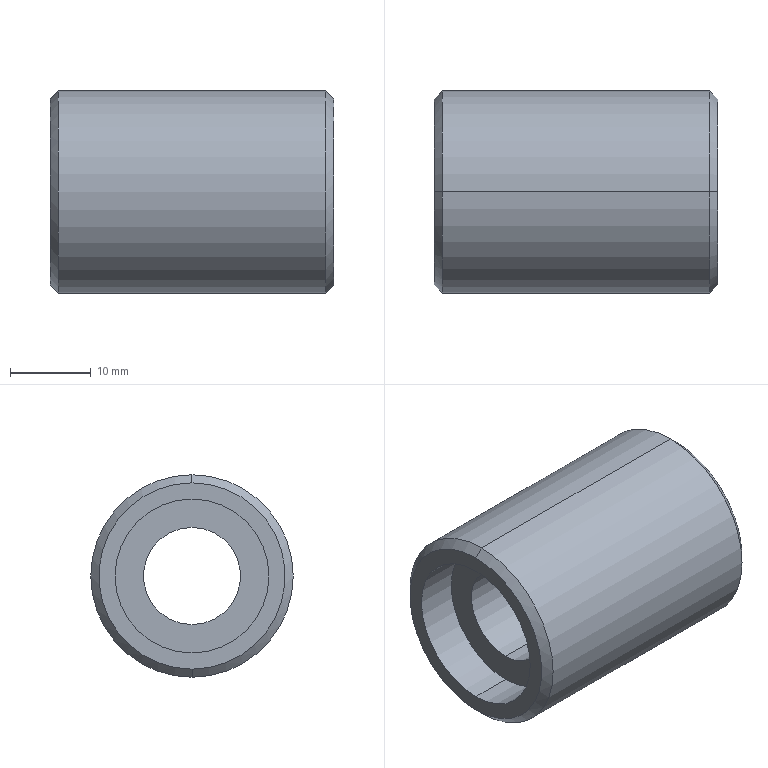Component | SolidWorks | CHEN123-AA-14-2 | 1 solid | 16 faces | box 35 x 25 x 25 mm | volume 11373 mm3 | cylinder 8 | cone 4 | plane 4 | commonest cylinder face diameters 19 x4 25 x2 12 x2
build123d program:
from build123d import *

# Parameters (mm, degrees)
SKETCH1_R           = 12.5
BOSS_EXTRUDE1_DEPTH = 17.5
SKETCH2_R           = 6
CUT_EXTRUDE1_DEPTH  = 40.211
SKETCH3_R           = 9.5
CUT_EXTRUDE2_DEPTH  = 5.2
CUT_EXTRUDE3_START  = -5.2
SKETCH4_R           = 9.5
CUT_EXTRUDE3_DEPTH  = 5.2
CHAMFER1_SIZE       = 1


with BuildPart() as part:
    # Sketch1 → Boss-Extrude1 (new, symmetric)
    with BuildSketch(Plane.XY):
        Circle(SKETCH1_R)
    extrude(amount=BOSS_EXTRUDE1_DEPTH, both=True)

    # Sketch2 → Cut-Extrude1 (cut, through all)
    with BuildSketch(Plane.XY.offset(17.5)):
        Circle(SKETCH2_R)
    extrude(amount=-CUT_EXTRUDE1_DEPTH, mode=Mode.SUBTRACT)

    # Sketch3 → Cut-Extrude2 (cut)
    with BuildSketch(Plane.XY.offset(17.5)):
        Circle(SKETCH3_R)
    extrude(amount=-CUT_EXTRUDE2_DEPTH, mode=Mode.SUBTRACT)

    # Sketch4 → Cut-Extrude3 (cut)
    with BuildSketch(Plane(origin=(0, 0, -17.5), x_dir=(-1, 0, 0), z_dir=(0, 0, -1)).offset(CUT_EXTRUDE3_START)):
        with Locations(Location((0, 0, 0), (0, 0, 180))):
            Circle(SKETCH4_R)
    extrude(amount=CUT_EXTRUDE3_DEPTH, mode=Mode.SUBTRACT)

    # Chamfer1
    chamfer1_edges = [part.edges().sort_by_distance(p)[0] for p in [
        (-12.5, 0, -17.5),
        (-12.5, 0, 17.5),
    ]]
    chamfer(chamfer1_edges, length=CHAMFER1_SIZE)


solid = part.part

# Placed as in the assembly
solid = solid.moved(Location((-0.0005, -45.999, -172), (0, 90, 0)))
STEP:
#1=COLOUR_RGB('',0.7922,0.8196,0.9333);
#2=FILL_AREA_STYLE_COLOUR('',#1);
#3=FILL_AREA_STYLE('',(#2));
#4=SURFACE_STYLE_FILL_AREA(#3);
#5=SURFACE_SIDE_STYLE('',(#4));
#6=SURFACE_STYLE_USAGE(.BOTH.,#5);
#7=PRESENTATION_STYLE_ASSIGNMENT((#6));
#8=CARTESIAN_POINT('',(0.689,-1.811,-7.224));
#9=VERTEX_POINT('',#8);
#10=CARTESIAN_POINT('',(0.689,-1.811,-6.319));
#11=VERTEX_POINT('',#10);
#12=CARTESIAN_POINT('',(0.689,-1.811,-6.772));
#13=DIRECTION('',(1.,0.,0.));
#14=DIRECTION('',(0.,0.,1.));
#15=AXIS2_PLACEMENT_3D('',#12,#13,#14);
#16=CIRCLE('',#15,0.4528);
#17=EDGE_CURVE('',#9,#11,#16,.T.);
#18=ORIENTED_EDGE('',*,*,#17,.F.);
#19=CARTESIAN_POINT('',(0.6496,-1.811,-7.264));
#20=VERTEX_POINT('',#19);
#21=CARTESIAN_POINT('',(0.6496,-1.811,-7.264));
#22=DIRECTION('',(-0.7071,-0.,-0.7071));
#23=VECTOR('',#22,39.37);
#24=LINE('',#21,#23);
#25=EDGE_CURVE('',#9,#20,#24,.T.);
#26=ORIENTED_EDGE('',*,*,#25,.T.);
#27=CARTESIAN_POINT('',(0.6496,-1.811,-6.28));
#28=VERTEX_POINT('',#27);
#29=CARTESIAN_POINT('',(0.6496,-1.811,-6.772));
#30=DIRECTION('',(-1.,0.,0.));
#31=DIRECTION('',(0.,0.,1.));
#32=AXIS2_PLACEMENT_3D('',#29,#30,#31);
#33=CIRCLE('',#32,0.4921);
#34=EDGE_CURVE('',#28,#20,#33,.T.);
#35=ORIENTED_EDGE('',*,*,#34,.F.);
#36=CARTESIAN_POINT('',(0.6496,-1.811,-6.28));
#37=DIRECTION('',(-0.7071,0.,0.7071));
#38=VECTOR('',#37,39.37);
#39=LINE('',#36,#38);
#40=EDGE_CURVE('',#11,#28,#39,.T.);
#41=ORIENTED_EDGE('',*,*,#40,.F.);
#42=EDGE_LOOP('',(#18,#26,#35,#41));
#43=FACE_OUTER_BOUND('',#42,.T.);
#44=CARTESIAN_POINT('',(0.6496,-1.811,-6.772));
#45=DIRECTION('',(-1.,0.,0.));
#46=DIRECTION('',(0.,0.,1.));
#47=AXIS2_PLACEMENT_3D('',#44,#45,#46);
#48=CONICAL_SURFACE('',#47,0.4921,0.7854);
#49=ADVANCED_FACE('',(#43),#48,.T.);
#50=CARTESIAN_POINT('',(-0.689,-1.811,-6.319));
#51=VERTEX_POINT('',#50);
#52=CARTESIAN_POINT('',(-0.689,-1.811,-7.224));
#53=VERTEX_POINT('',#52);
#54=CARTESIAN_POINT('',(-0.689,-1.811,-6.772));
#55=DIRECTION('',(-1.,0.,0.));
#56=DIRECTION('',(0.,0.,1.));
#57=AXIS2_PLACEMENT_3D('',#54,#55,#56);
#58=CIRCLE('',#57,0.4528);
#59=EDGE_CURVE('',#51,#53,#58,.T.);
#60=ORIENTED_EDGE('',*,*,#59,.F.);
#61=CARTESIAN_POINT('',(-0.6496,-1.811,-6.28));
#62=VERTEX_POINT('',#61);
#63=CARTESIAN_POINT('',(-0.689,-1.811,-6.319));
#64=DIRECTION('',(0.7071,0.,0.7071));
#65=VECTOR('',#64,39.37);
#66=LINE('',#63,#65);
#67=EDGE_CURVE('',#51,#62,#66,.T.);
#68=ORIENTED_EDGE('',*,*,#67,.T.);
#69=CARTESIAN_POINT('',(-0.6496,-1.811,-7.264));
#70=VERTEX_POINT('',#69);
#71=CARTESIAN_POINT('',(-0.6496,-1.811,-6.772));
#72=DIRECTION('',(1.,0.,0.));
#73=DIRECTION('',(0.,0.,1.));
#74=AXIS2_PLACEMENT_3D('',#71,#72,#73);
#75=CIRCLE('',#74,0.4921);
#76=EDGE_CURVE('',#70,#62,#75,.T.);
#77=ORIENTED_EDGE('',*,*,#76,.F.);
#78=CARTESIAN_POINT('',(-0.689,-1.811,-7.224));
#79=DIRECTION('',(0.7071,-0.,-0.7071));
#80=VECTOR('',#79,39.37);
#81=LINE('',#78,#80);
#82=EDGE_CURVE('',#53,#70,#81,.T.);
#83=ORIENTED_EDGE('',*,*,#82,.F.);
#84=EDGE_LOOP('',(#60,#68,#77,#83));
#85=FACE_OUTER_BOUND('',#84,.T.);
#86=CARTESIAN_POINT('',(-0.689,-1.811,-6.772));
#87=DIRECTION('',(1.,0.,0.));
#88=DIRECTION('',(0.,-0.,-1.));
#89=AXIS2_PLACEMENT_3D('',#86,#87,#88);
#90=CONICAL_SURFACE('',#89,0.4528,0.7854);
#91=ADVANCED_FACE('',(#85),#90,.T.);
#92=CARTESIAN_POINT('',(0.4842,-1.811,-6.398));
#93=VERTEX_POINT('',#92);
#94=CARTESIAN_POINT('',(0.4842,-1.811,-7.146));
#95=VERTEX_POINT('',#94);
#96=CARTESIAN_POINT('',(0.4842,-1.811,-6.772));
#97=DIRECTION('',(1.,0.,0.));
#98=DIRECTION('',(0.,0.,-1.));
#99=AXIS2_PLACEMENT_3D('',#96,#97,#98);
#100=CIRCLE('',#99,0.374);
#101=EDGE_CURVE('',#93,#95,#100,.T.);
#102=ORIENTED_EDGE('',*,*,#101,.F.);
#103=CARTESIAN_POINT('',(0.689,-1.811,-6.398));
#104=VERTEX_POINT('',#103);
#105=CARTESIAN_POINT('',(0.4842,-1.811,-6.398));
#106=DIRECTION('',(1.,0.,0.));
#107=VECTOR('',#106,39.37);
#108=LINE('',#105,#107);
#109=EDGE_CURVE('',#93,#104,#108,.T.);
#110=ORIENTED_EDGE('',*,*,#109,.T.);
#111=CARTESIAN_POINT('',(0.689,-1.811,-7.146));
#112=VERTEX_POINT('',#111);
#113=CARTESIAN_POINT('',(0.689,-1.811,-6.772));
#114=DIRECTION('',(1.,0.,0.));
#115=DIRECTION('',(0.,0.,-1.));
#116=AXIS2_PLACEMENT_3D('',#113,#114,#115);
#117=CIRCLE('',#116,0.374);
#118=EDGE_CURVE('',#104,#112,#117,.T.);
#119=ORIENTED_EDGE('',*,*,#118,.T.);
#120=CARTESIAN_POINT('',(0.4842,-1.811,-7.146));
#121=DIRECTION('',(1.,0.,0.));
#122=VECTOR('',#121,39.37);
#123=LINE('',#120,#122);
#124=EDGE_CURVE('',#95,#112,#123,.T.);
#125=ORIENTED_EDGE('',*,*,#124,.F.);
#126=EDGE_LOOP('',(#102,#110,#119,#125));
#127=FACE_OUTER_BOUND('',#126,.T.);
#128=CARTESIAN_POINT('',(0.4842,-1.811,-6.772));
#129=DIRECTION('',(1.,0.,0.));
#130=DIRECTION('',(0.,0.,-1.));
#131=AXIS2_PLACEMENT_3D('',#128,#129,#130);
#132=CYLINDRICAL_SURFACE('',#131,0.374);
#133=ADVANCED_FACE('',(#127),#132,.F.);
#134=CARTESIAN_POINT('',(-0.4843,-1.811,-7.146));
#135=VERTEX_POINT('',#134);
#136=CARTESIAN_POINT('',(-0.4843,-1.811,-6.398));
#137=VERTEX_POINT('',#136);
#138=CARTESIAN_POINT('',(-0.4843,-1.811,-6.772));
#139=DIRECTION('',(-1.,0.,0.));
#140=DIRECTION('',(0.,0.,1.));
#141=AXIS2_PLACEMENT_3D('',#138,#139,#140);
#142=CIRCLE('',#141,0.374);
#143=EDGE_CURVE('',#135,#137,#142,.T.);
#144=ORIENTED_EDGE('',*,*,#143,.F.);
#145=CARTESIAN_POINT('',(-0.689,-1.811,-7.146));
#146=VERTEX_POINT('',#145);
#147=CARTESIAN_POINT('',(-0.4843,-1.811,-7.146));
#148=DIRECTION('',(-1.,0.,0.));
#149=VECTOR('',#148,39.37);
#150=LINE('',#147,#149);
#151=EDGE_CURVE('',#135,#146,#150,.T.);
#152=ORIENTED_EDGE('',*,*,#151,.T.);
#153=CARTESIAN_POINT('',(-0.689,-1.811,-6.398));
#154=VERTEX_POINT('',#153);
#155=CARTESIAN_POINT('',(-0.689,-1.811,-6.772));
#156=DIRECTION('',(-1.,0.,0.));
#157=DIRECTION('',(0.,0.,1.));
#158=AXIS2_PLACEMENT_3D('',#155,#156,#157);
#159=CIRCLE('',#158,0.374);
#160=EDGE_CURVE('',#146,#154,#159,.T.);
#161=ORIENTED_EDGE('',*,*,#160,.T.);
#162=CARTESIAN_POINT('',(-0.4843,-1.811,-6.398));
#163=DIRECTION('',(-1.,0.,0.));
#164=VECTOR('',#163,39.37);
#165=LINE('',#162,#164);
#166=EDGE_CURVE('',#137,#154,#165,.T.);
#167=ORIENTED_EDGE('',*,*,#166,.F.);
#168=EDGE_LOOP('',(#144,#152,#161,#167));
#169=FACE_OUTER_BOUND('',#168,.T.);
#170=CARTESIAN_POINT('',(-0.4843,-1.811,-6.772));
#171=DIRECTION('',(-1.,0.,0.));
#172=DIRECTION('',(0.,0.,1.));
#173=AXIS2_PLACEMENT_3D('',#170,#171,#172);
#174=CYLINDRICAL_SURFACE('',#173,0.374);
#175=ADVANCED_FACE('',(#169),#174,.F.);
#176=ORIENTED_EDGE('',*,*,#76,.T.);
#177=CARTESIAN_POINT('',(-0.689,-1.811,-6.28));
#178=DIRECTION('',(1.,0.,0.));
#179=VECTOR('',#178,39.37);
#180=LINE('',#177,#179);
#181=EDGE_CURVE('',#62,#28,#180,.T.);
#182=ORIENTED_EDGE('',*,*,#181,.T.);
#183=ORIENTED_EDGE('',*,*,#34,.T.);
#184=CARTESIAN_POINT('',(-0.689,-1.811,-7.264));
#185=DIRECTION('',(1.,0.,0.));
#186=VECTOR('',#185,39.37);
#187=LINE('',#184,#186);
#188=EDGE_CURVE('',#70,#20,#187,.T.);
#189=ORIENTED_EDGE('',*,*,#188,.F.);
#190=EDGE_LOOP('',(#176,#182,#183,#189));
#191=FACE_OUTER_BOUND('',#190,.T.);
#192=CARTESIAN_POINT('',(-0.689,-1.811,-6.772));
#193=DIRECTION('',(1.,0.,0.));
#194=DIRECTION('',(0.,-0.,-1.));
#195=AXIS2_PLACEMENT_3D('',#192,#193,#194);
#196=CYLINDRICAL_SURFACE('',#195,0.4921);
#197=ADVANCED_FACE('',(#191),#196,.T.);
#198=CARTESIAN_POINT('',(0.4842,-1.811,-7.008));
#199=VERTEX_POINT('',#198);
#200=CARTESIAN_POINT('',(0.4842,-1.811,-6.535));
#201=VERTEX_POINT('',#200);
#202=CARTESIAN_POINT('',(0.4842,-1.811,-6.772));
#203=DIRECTION('',(-1.,0.,0.));
#204=DIRECTION('',(0.,0.,-1.));
#205=AXIS2_PLACEMENT_3D('',#202,#203,#204);
#206=CIRCLE('',#205,0.2362);
#207=EDGE_CURVE('',#199,#201,#206,.T.);
#208=ORIENTED_EDGE('',*,*,#207,.F.);
#209=CARTESIAN_POINT('',(-0.4843,-1.811,-7.008));
#210=VERTEX_POINT('',#209);
#211=CARTESIAN_POINT('',(0.689,-1.811,-7.008));
#212=DIRECTION('',(-1.,0.,0.));
#213=VECTOR('',#212,39.37);
#214=LINE('',#211,#213);
#215=EDGE_CURVE('',#199,#210,#214,.T.);
#216=ORIENTED_EDGE('',*,*,#215,.T.);
#217=CARTESIAN_POINT('',(-0.4843,-1.811,-6.535));
#218=VERTEX_POINT('',#217);
#219=CARTESIAN_POINT('',(-0.4843,-1.811,-6.772));
#220=DIRECTION('',(1.,0.,0.));
#221=DIRECTION('',(0.,0.,1.));
#222=AXIS2_PLACEMENT_3D('',#219,#220,#221);
#223=CIRCLE('',#222,0.2362);
#224=EDGE_CURVE('',#218,#210,#223,.T.);
#225=ORIENTED_EDGE('',*,*,#224,.F.);
#226=CARTESIAN_POINT('',(0.689,-1.811,-6.535));
#227=DIRECTION('',(-1.,0.,0.));
#228=VECTOR('',#227,39.37);
#229=LINE('',#226,#228);
#230=EDGE_CURVE('',#201,#218,#229,.T.);
#231=ORIENTED_EDGE('',*,*,#230,.F.);
#232=EDGE_LOOP('',(#208,#216,#225,#231));
#233=FACE_OUTER_BOUND('',#232,.T.);
#234=CARTESIAN_POINT('',(0.689,-1.811,-6.772));
#235=DIRECTION('',(-1.,0.,0.));
#236=DIRECTION('',(0.,0.,1.));
#237=AXIS2_PLACEMENT_3D('',#234,#235,#236);
#238=CYLINDRICAL_SURFACE('',#237,0.2362);
#239=ADVANCED_FACE('',(#233),#238,.F.);
#240=ORIENTED_EDGE('',*,*,#215,.F.);
#241=CARTESIAN_POINT('',(0.4842,-1.811,-6.772));
#242=DIRECTION('',(-1.,0.,0.));
#243=DIRECTION('',(0.,0.,-1.));
#244=AXIS2_PLACEMENT_3D('',#241,#242,#243);
#245=CIRCLE('',#244,0.2362);
#246=EDGE_CURVE('',#201,#199,#245,.T.);
#247=ORIENTED_EDGE('',*,*,#246,.F.);
#248=ORIENTED_EDGE('',*,*,#230,.T.);
#249=CARTESIAN_POINT('',(-0.4843,-1.811,-6.772));
#250=DIRECTION('',(1.,0.,0.));
#251=DIRECTION('',(0.,0.,1.));
#252=AXIS2_PLACEMENT_3D('',#249,#250,#251);
#253=CIRCLE('',#252,0.2362);
#254=EDGE_CURVE('',#210,#218,#253,.T.);
#255=ORIENTED_EDGE('',*,*,#254,.F.);
#256=EDGE_LOOP('',(#240,#247,#248,#255));
#257=FACE_OUTER_BOUND('',#256,.T.);
#258=CARTESIAN_POINT('',(0.689,-1.811,-6.772));
#259=DIRECTION('',(-1.,0.,0.));
#260=DIRECTION('',(0.,0.,1.));
#261=AXIS2_PLACEMENT_3D('',#258,#259,#260);
#262=CYLINDRICAL_SURFACE('',#261,0.2362);
#263=ADVANCED_FACE('',(#257),#262,.F.);
#264=ORIENTED_EDGE('',*,*,#181,.F.);
#265=CARTESIAN_POINT('',(-0.6496,-1.811,-6.772));
#266=DIRECTION('',(1.,0.,0.));
#267=DIRECTION('',(0.,0.,1.));
#268=AXIS2_PLACEMENT_3D('',#265,#266,#267);
#269=CIRCLE('',#268,0.4921);
#270=EDGE_CURVE('',#62,#70,#269,.T.);
#271=ORIENTED_EDGE('',*,*,#270,.T.);
#272=ORIENTED_EDGE('',*,*,#188,.T.);
#273=CARTESIAN_POINT('',(0.6496,-1.811,-6.772));
#274=DIRECTION('',(-1.,0.,0.));
#275=DIRECTION('',(0.,0.,1.));
#276=AXIS2_PLACEMENT_3D('',#273,#274,#275);
#277=CIRCLE('',#276,0.4921);
#278=EDGE_CURVE('',#20,#28,#277,.T.);
#279=ORIENTED_EDGE('',*,*,#278,.T.);
#280=EDGE_LOOP('',(#264,#271,#272,#279));
#281=FACE_OUTER_BOUND('',#280,.T.);
#282=CARTESIAN_POINT('',(-0.689,-1.811,-6.772));
#283=DIRECTION('',(1.,0.,0.));
#284=DIRECTION('',(0.,-0.,-1.));
#285=AXIS2_PLACEMENT_3D('',#282,#283,#284);
#286=CYLINDRICAL_SURFACE('',#285,0.4921);
#287=ADVANCED_FACE('',(#281),#286,.T.);
#288=CARTESIAN_POINT('',(-0.689,-1.811,-6.772));
#289=DIRECTION('',(-1.,0.,0.));
#290=DIRECTION('',(0.,0.,1.));
#291=AXIS2_PLACEMENT_3D('',#288,#289,#290);
#292=CIRCLE('',#291,0.4528);
#293=EDGE_CURVE('',#53,#51,#292,.T.);
#294=ORIENTED_EDGE('',*,*,#293,.T.);
#295=ORIENTED_EDGE('',*,*,#59,.T.);
#296=EDGE_LOOP('',(#294,#295));
#297=FACE_OUTER_BOUND('',#296,.T.);
#298=CARTESIAN_POINT('',(-0.689,-1.811,-6.772));
#299=DIRECTION('',(-1.,0.,0.));
#300=DIRECTION('',(0.,0.,1.));
#301=AXIS2_PLACEMENT_3D('',#298,#299,#300);
#302=CIRCLE('',#301,0.374);
#303=EDGE_CURVE('',#154,#146,#302,.T.);
#304=ORIENTED_EDGE('',*,*,#303,.F.);
#305=ORIENTED_EDGE('',*,*,#160,.F.);
#306=EDGE_LOOP('',(#304,#305));
#307=FACE_BOUND('',#306,.T.);
#308=CARTESIAN_POINT('',(-0.689,-1.811,-6.772));
#309=DIRECTION('',(-1.,0.,0.));
#310=DIRECTION('',(0.,0.,1.));
#311=AXIS2_PLACEMENT_3D('',#308,#309,#310);
#312=PLANE('',#311);
#313=ADVANCED_FACE('',(#297,#307),#312,.T.);
#314=CARTESIAN_POINT('',(0.689,-1.811,-6.772));
#315=DIRECTION('',(1.,0.,0.));
#316=DIRECTION('',(0.,0.,1.));
#317=AXIS2_PLACEMENT_3D('',#314,#315,#316);
#318=CIRCLE('',#317,0.4528);
#319=EDGE_CURVE('',#11,#9,#318,.T.);
#320=ORIENTED_EDGE('',*,*,#319,.T.);
#321=ORIENTED_EDGE('',*,*,#17,.T.);
#322=EDGE_LOOP('',(#320,#321));
#323=FACE_OUTER_BOUND('',#322,.T.);
#324=CARTESIAN_POINT('',(0.689,-1.811,-6.772));
#325=DIRECTION('',(1.,0.,0.));
#326=DIRECTION('',(0.,0.,-1.));
#327=AXIS2_PLACEMENT_3D('',#324,#325,#326);
#328=CIRCLE('',#327,0.374);
#329=EDGE_CURVE('',#112,#104,#328,.T.);
#330=ORIENTED_EDGE('',*,*,#329,.F.);
#331=ORIENTED_EDGE('',*,*,#118,.F.);
#332=EDGE_LOOP('',(#330,#331));
#333=FACE_BOUND('',#332,.T.);
#334=CARTESIAN_POINT('',(0.689,-1.811,-6.772));
#335=DIRECTION('',(-1.,0.,0.));
#336=DIRECTION('',(0.,0.,1.));
#337=AXIS2_PLACEMENT_3D('',#334,#335,#336);
#338=PLANE('',#337);
#339=ADVANCED_FACE('',(#323,#333),#338,.F.);
#340=CARTESIAN_POINT('',(-0.4843,-1.811,-6.772));
#341=DIRECTION('',(-1.,0.,0.));
#342=DIRECTION('',(0.,0.,1.));
#343=AXIS2_PLACEMENT_3D('',#340,#341,#342);
#344=CIRCLE('',#343,0.374);
#345=EDGE_CURVE('',#137,#135,#344,.T.);
#346=ORIENTED_EDGE('',*,*,#345,.T.);
#347=ORIENTED_EDGE('',*,*,#143,.T.);
#348=EDGE_LOOP('',(#346,#347));
#349=FACE_OUTER_BOUND('',#348,.T.);
#350=ORIENTED_EDGE('',*,*,#224,.T.);
#351=ORIENTED_EDGE('',*,*,#254,.T.);
#352=EDGE_LOOP('',(#350,#351));
#353=FACE_BOUND('',#352,.T.);
#354=CARTESIAN_POINT('',(-0.4843,-1.811,-6.772));
#355=DIRECTION('',(-1.,0.,0.));
#356=DIRECTION('',(0.,0.,1.));
#357=AXIS2_PLACEMENT_3D('',#354,#355,#356);
#358=PLANE('',#357);
#359=ADVANCED_FACE('',(#349,#353),#358,.T.);
#360=ORIENTED_EDGE('',*,*,#151,.F.);
#361=ORIENTED_EDGE('',*,*,#345,.F.);
#362=ORIENTED_EDGE('',*,*,#166,.T.);
#363=ORIENTED_EDGE('',*,*,#303,.T.);
#364=EDGE_LOOP('',(#360,#361,#362,#363));
#365=FACE_OUTER_BOUND('',#364,.T.);
#366=CARTESIAN_POINT('',(-0.4843,-1.811,-6.772));
#367=DIRECTION('',(-1.,0.,0.));
#368=DIRECTION('',(0.,0.,1.));
#369=AXIS2_PLACEMENT_3D('',#366,#367,#368);
#370=CYLINDRICAL_SURFACE('',#369,0.374);
#371=ADVANCED_FACE('',(#365),#370,.F.);
#372=CARTESIAN_POINT('',(0.4842,-1.811,-6.772));
#373=DIRECTION('',(1.,0.,0.));
#374=DIRECTION('',(0.,0.,-1.));
#375=AXIS2_PLACEMENT_3D('',#372,#373,#374);
#376=CIRCLE('',#375,0.374);
#377=EDGE_CURVE('',#95,#93,#376,.T.);
#378=ORIENTED_EDGE('',*,*,#377,.T.);
#379=ORIENTED_EDGE('',*,*,#101,.T.);
#380=EDGE_LOOP('',(#378,#379));
#381=FACE_OUTER_BOUND('',#380,.T.);
#382=ORIENTED_EDGE('',*,*,#246,.T.);
#383=ORIENTED_EDGE('',*,*,#207,.T.);
#384=EDGE_LOOP('',(#382,#383));
#385=FACE_BOUND('',#384,.T.);
#386=CARTESIAN_POINT('',(0.4842,-1.811,-6.772));
#387=DIRECTION('',(1.,0.,0.));
#388=DIRECTION('',(0.,-0.,-1.));
#389=AXIS2_PLACEMENT_3D('',#386,#387,#388);
#390=PLANE('',#389);
#391=ADVANCED_FACE('',(#381,#385),#390,.T.);
#392=ORIENTED_EDGE('',*,*,#109,.F.);
#393=ORIENTED_EDGE('',*,*,#377,.F.);
#394=ORIENTED_EDGE('',*,*,#124,.T.);
#395=ORIENTED_EDGE('',*,*,#329,.T.);
#396=EDGE_LOOP('',(#392,#393,#394,#395));
#397=FACE_OUTER_BOUND('',#396,.T.);
#398=CARTESIAN_POINT('',(0.4842,-1.811,-6.772));
#399=DIRECTION('',(1.,0.,0.));
#400=DIRECTION('',(0.,0.,-1.));
#401=AXIS2_PLACEMENT_3D('',#398,#399,#400);
#402=CYLINDRICAL_SURFACE('',#401,0.374);
#403=ADVANCED_FACE('',(#397),#402,.F.);
#404=ORIENTED_EDGE('',*,*,#67,.F.);
#405=ORIENTED_EDGE('',*,*,#293,.F.);
#406=ORIENTED_EDGE('',*,*,#82,.T.);
#407=ORIENTED_EDGE('',*,*,#270,.F.);
#408=EDGE_LOOP('',(#404,#405,#406,#407));
#409=FACE_OUTER_BOUND('',#408,.T.);
#410=CARTESIAN_POINT('',(-0.689,-1.811,-6.772));
#411=DIRECTION('',(1.,0.,0.));
#412=DIRECTION('',(0.,-0.,-1.));
#413=AXIS2_PLACEMENT_3D('',#410,#411,#412);
#414=CONICAL_SURFACE('',#413,0.4528,0.7854);
#415=ADVANCED_FACE('',(#409),#414,.T.);
#416=ORIENTED_EDGE('',*,*,#25,.F.);
#417=ORIENTED_EDGE('',*,*,#319,.F.);
#418=ORIENTED_EDGE('',*,*,#40,.T.);
#419=ORIENTED_EDGE('',*,*,#278,.F.);
#420=EDGE_LOOP('',(#416,#417,#418,#419));
#421=FACE_OUTER_BOUND('',#420,.T.);
#422=CARTESIAN_POINT('',(0.6496,-1.811,-6.772));
#423=DIRECTION('',(-1.,0.,0.));
#424=DIRECTION('',(0.,0.,1.));
#425=AXIS2_PLACEMENT_3D('',#422,#423,#424);
#426=CONICAL_SURFACE('',#425,0.4921,0.7854);
#427=ADVANCED_FACE('',(#421),#426,.T.);
#428=CLOSED_SHELL('',(#49,#91,#133,#175,#197,#239,#263,#287,#313,#339,#359,#371,#391,#403,#415,#427));
#429=MANIFOLD_SOLID_BREP('',#428);
#430=STYLED_ITEM('',(#7),#429);
#431=(LENGTH_UNIT()NAMED_UNIT(*)SI_UNIT($,.METRE.));
#432=LENGTH_MEASURE_WITH_UNIT(LENGTH_MEASURE(0.0254),#431);
#433=DIMENSIONAL_EXPONENTS(1.,0.,0.,0.,0.,0.,0.);
#434=(CONVERSION_BASED_UNIT('',#432)LENGTH_UNIT()NAMED_UNIT(#433));
#435=UNCERTAINTY_MEASURE_WITH_UNIT(LENGTH_MEASURE(0.00001),#434,'','');
#436=(NAMED_UNIT(*)PLANE_ANGLE_UNIT()SI_UNIT($,.RADIAN.));
#437=(NAMED_UNIT(*)SI_UNIT($,.STERADIAN.)SOLID_ANGLE_UNIT());
#438=(GEOMETRIC_REPRESENTATION_CONTEXT(3)GLOBAL_UNCERTAINTY_ASSIGNED_CONTEXT((#435))GLOBAL_UNIT_ASSIGNED_CONTEXT((#434,#436,#437))REPRESENTATION_CONTEXT('',''));
#439=MECHANICAL_DESIGN_GEOMETRIC_PRESENTATION_REPRESENTATION('',(#430),#438);
#440=PRESENTATION_LAYER_ASSIGNMENT('','',(#430));
#441=CARTESIAN_POINT('',(0.,0.,0.));
#442=DIRECTION('',(0.,0.,1.));
#443=DIRECTION('',(1.,0.,0.));
#444=AXIS2_PLACEMENT_3D('',#441,#442,#443);
#445=(LENGTH_UNIT()NAMED_UNIT(*)SI_UNIT($,.METRE.));
#446=LENGTH_MEASURE_WITH_UNIT(LENGTH_MEASURE(0.0254),#445);
#447=DIMENSIONAL_EXPONENTS(1.,0.,0.,0.,0.,0.,0.);
#448=(CONVERSION_BASED_UNIT('',#446)LENGTH_UNIT()NAMED_UNIT(#447));
#449=UNCERTAINTY_MEASURE_WITH_UNIT(LENGTH_MEASURE(0.00001),#448,'','');
#450=(NAMED_UNIT(*)PLANE_ANGLE_UNIT()SI_UNIT($,.RADIAN.));
#451=(NAMED_UNIT(*)SI_UNIT($,.STERADIAN.)SOLID_ANGLE_UNIT());
#452=(GEOMETRIC_REPRESENTATION_CONTEXT(3)GLOBAL_UNCERTAINTY_ASSIGNED_CONTEXT((#449))GLOBAL_UNIT_ASSIGNED_CONTEXT((#448,#450,#451))REPRESENTATION_CONTEXT('',''));
#453=ADVANCED_BREP_SHAPE_REPRESENTATION('',(#429,#444),#452);